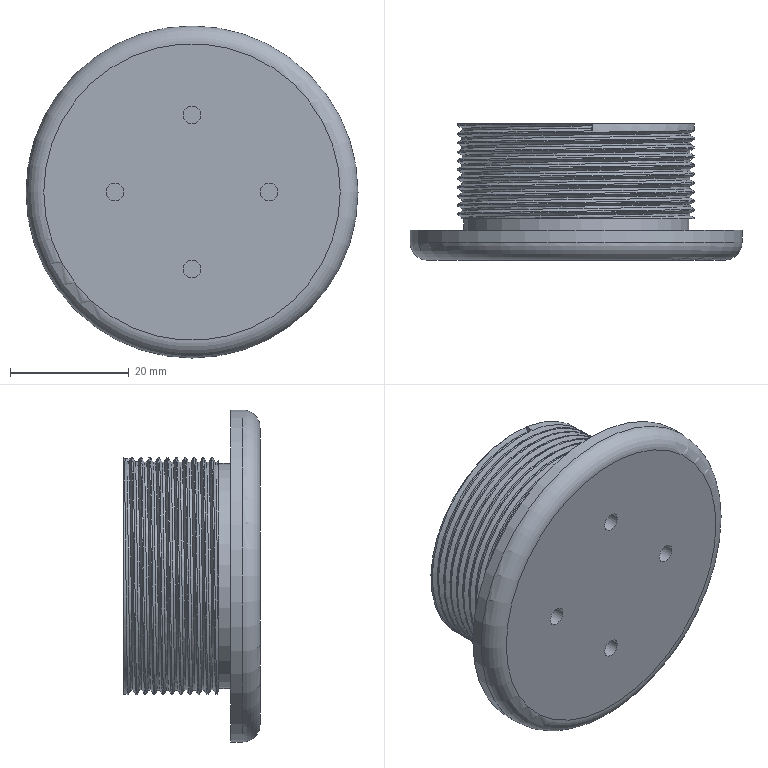Component | NX | 10 | 1 solid | 24 faces | volume 21152 mm3 | plane 11 | cylinder 10 | spline 2 | torus 1 | commonest cylinder face diameters 3 x4 40 x1 38 x1 56 x1 35 x1 24 x1 38.5 x1